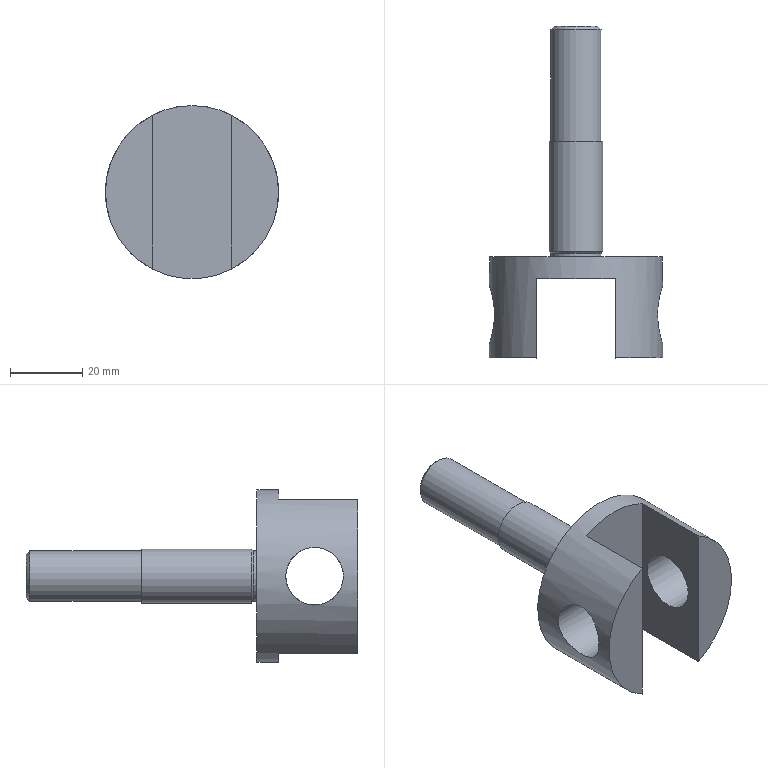Component | NX | ROTOR_SHAFT | 1 solid | 19 faces | volume 33682 mm3 | plane 9 | cylinder 6 | cone 4 | commonest cylinder face diameters 16 x2 14 x2 48 x1 15 x1